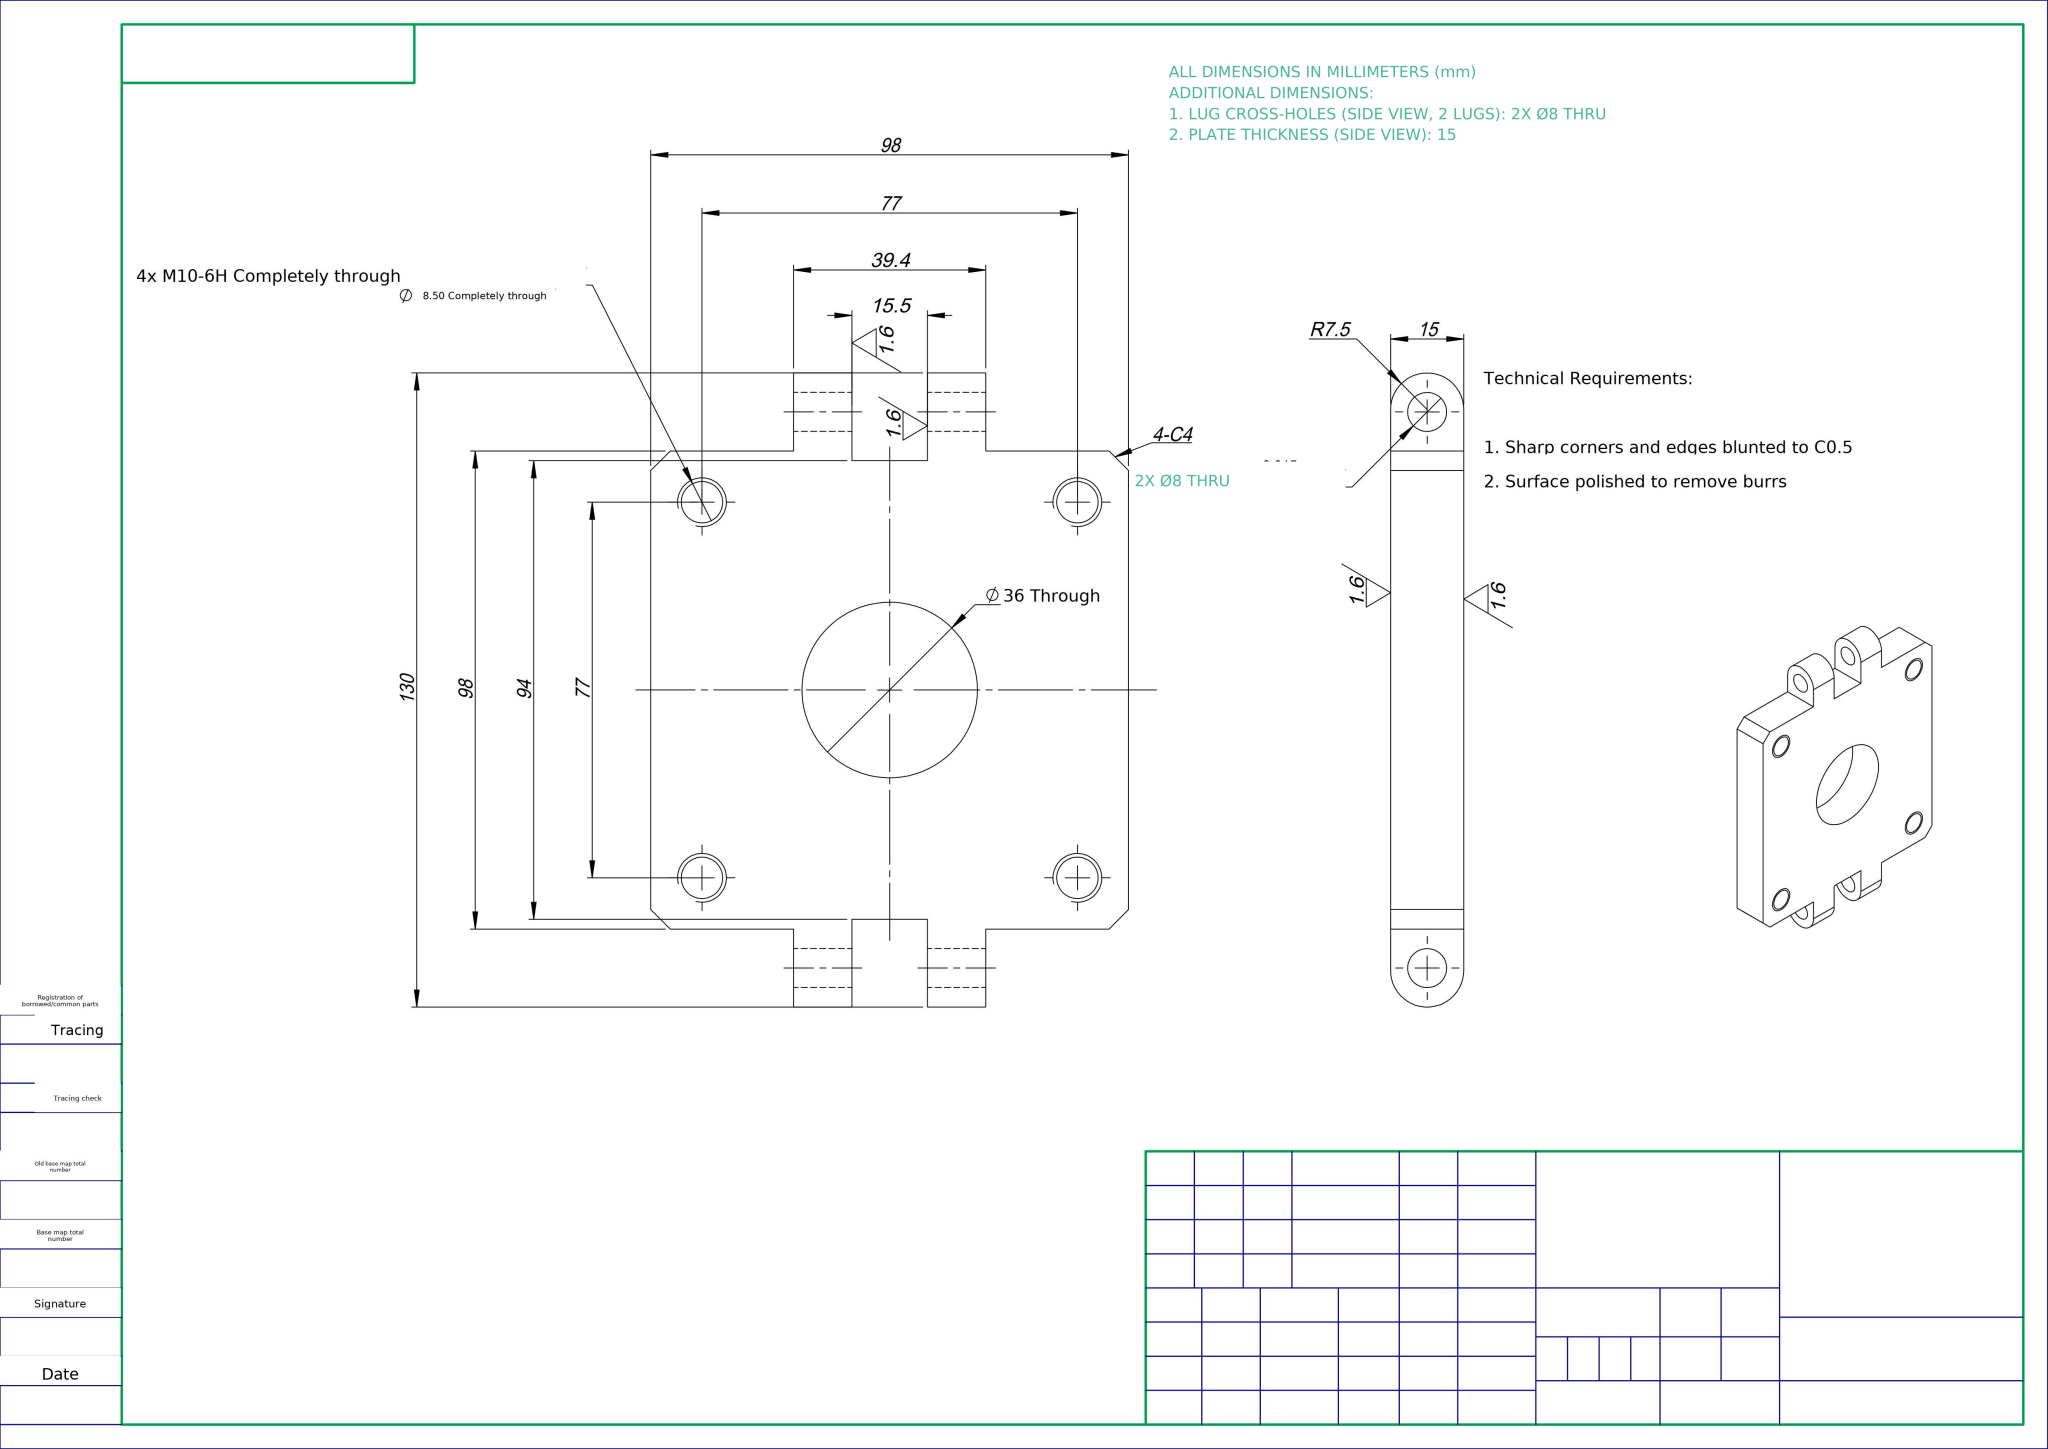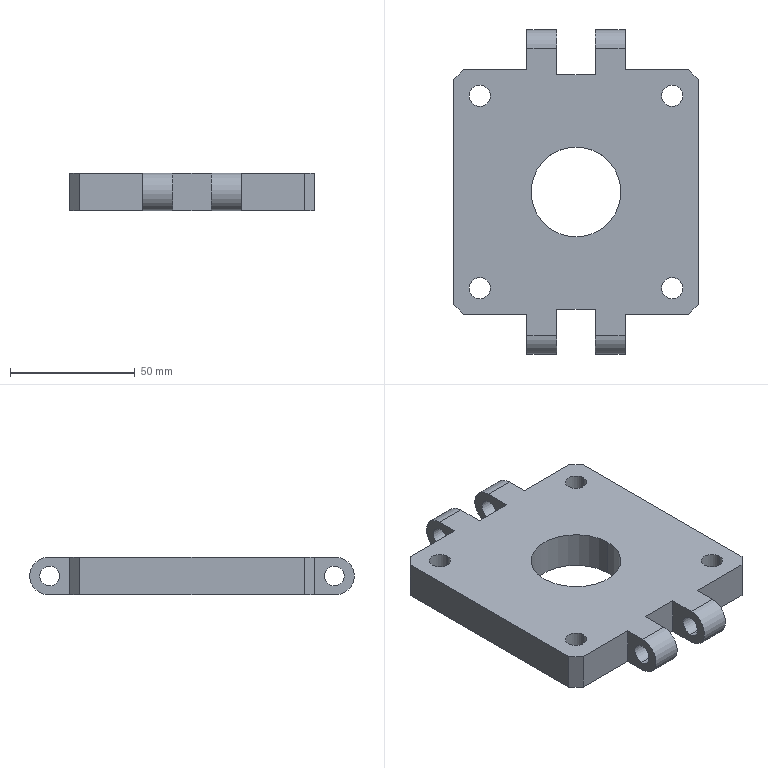Part | NX | mm | 1 solid | 44 faces | box 98 x 130 x 15 mm | volume 131892 mm3 | cylinder 22 | plane 22 | commonest cylinder face diameters 8 x8 8.5 x8 15 x4 36 x2